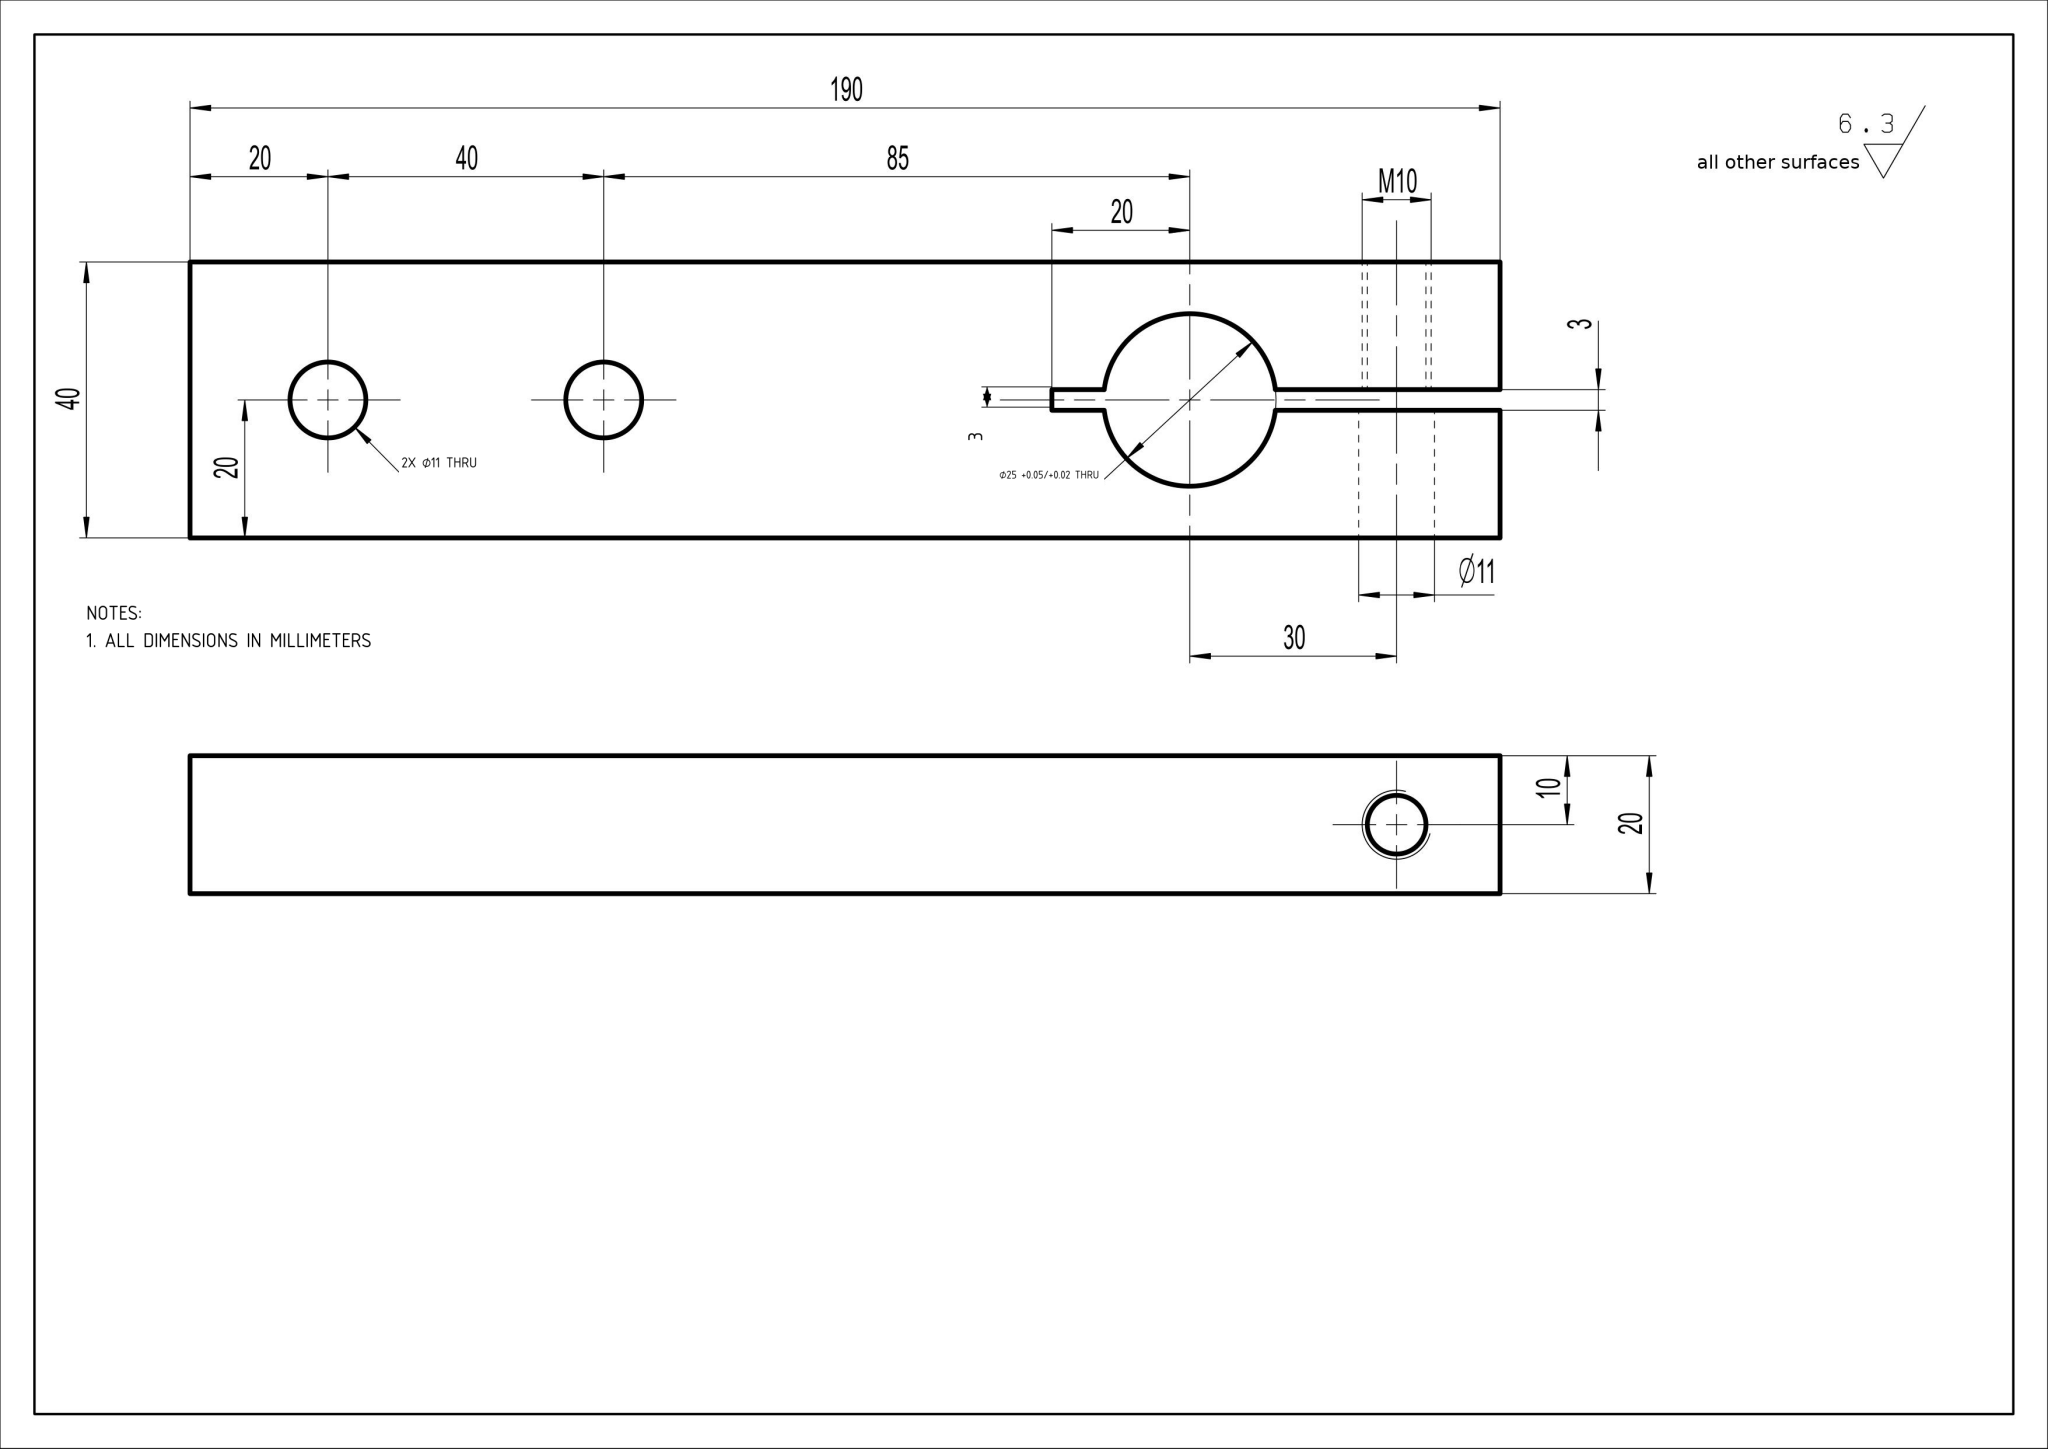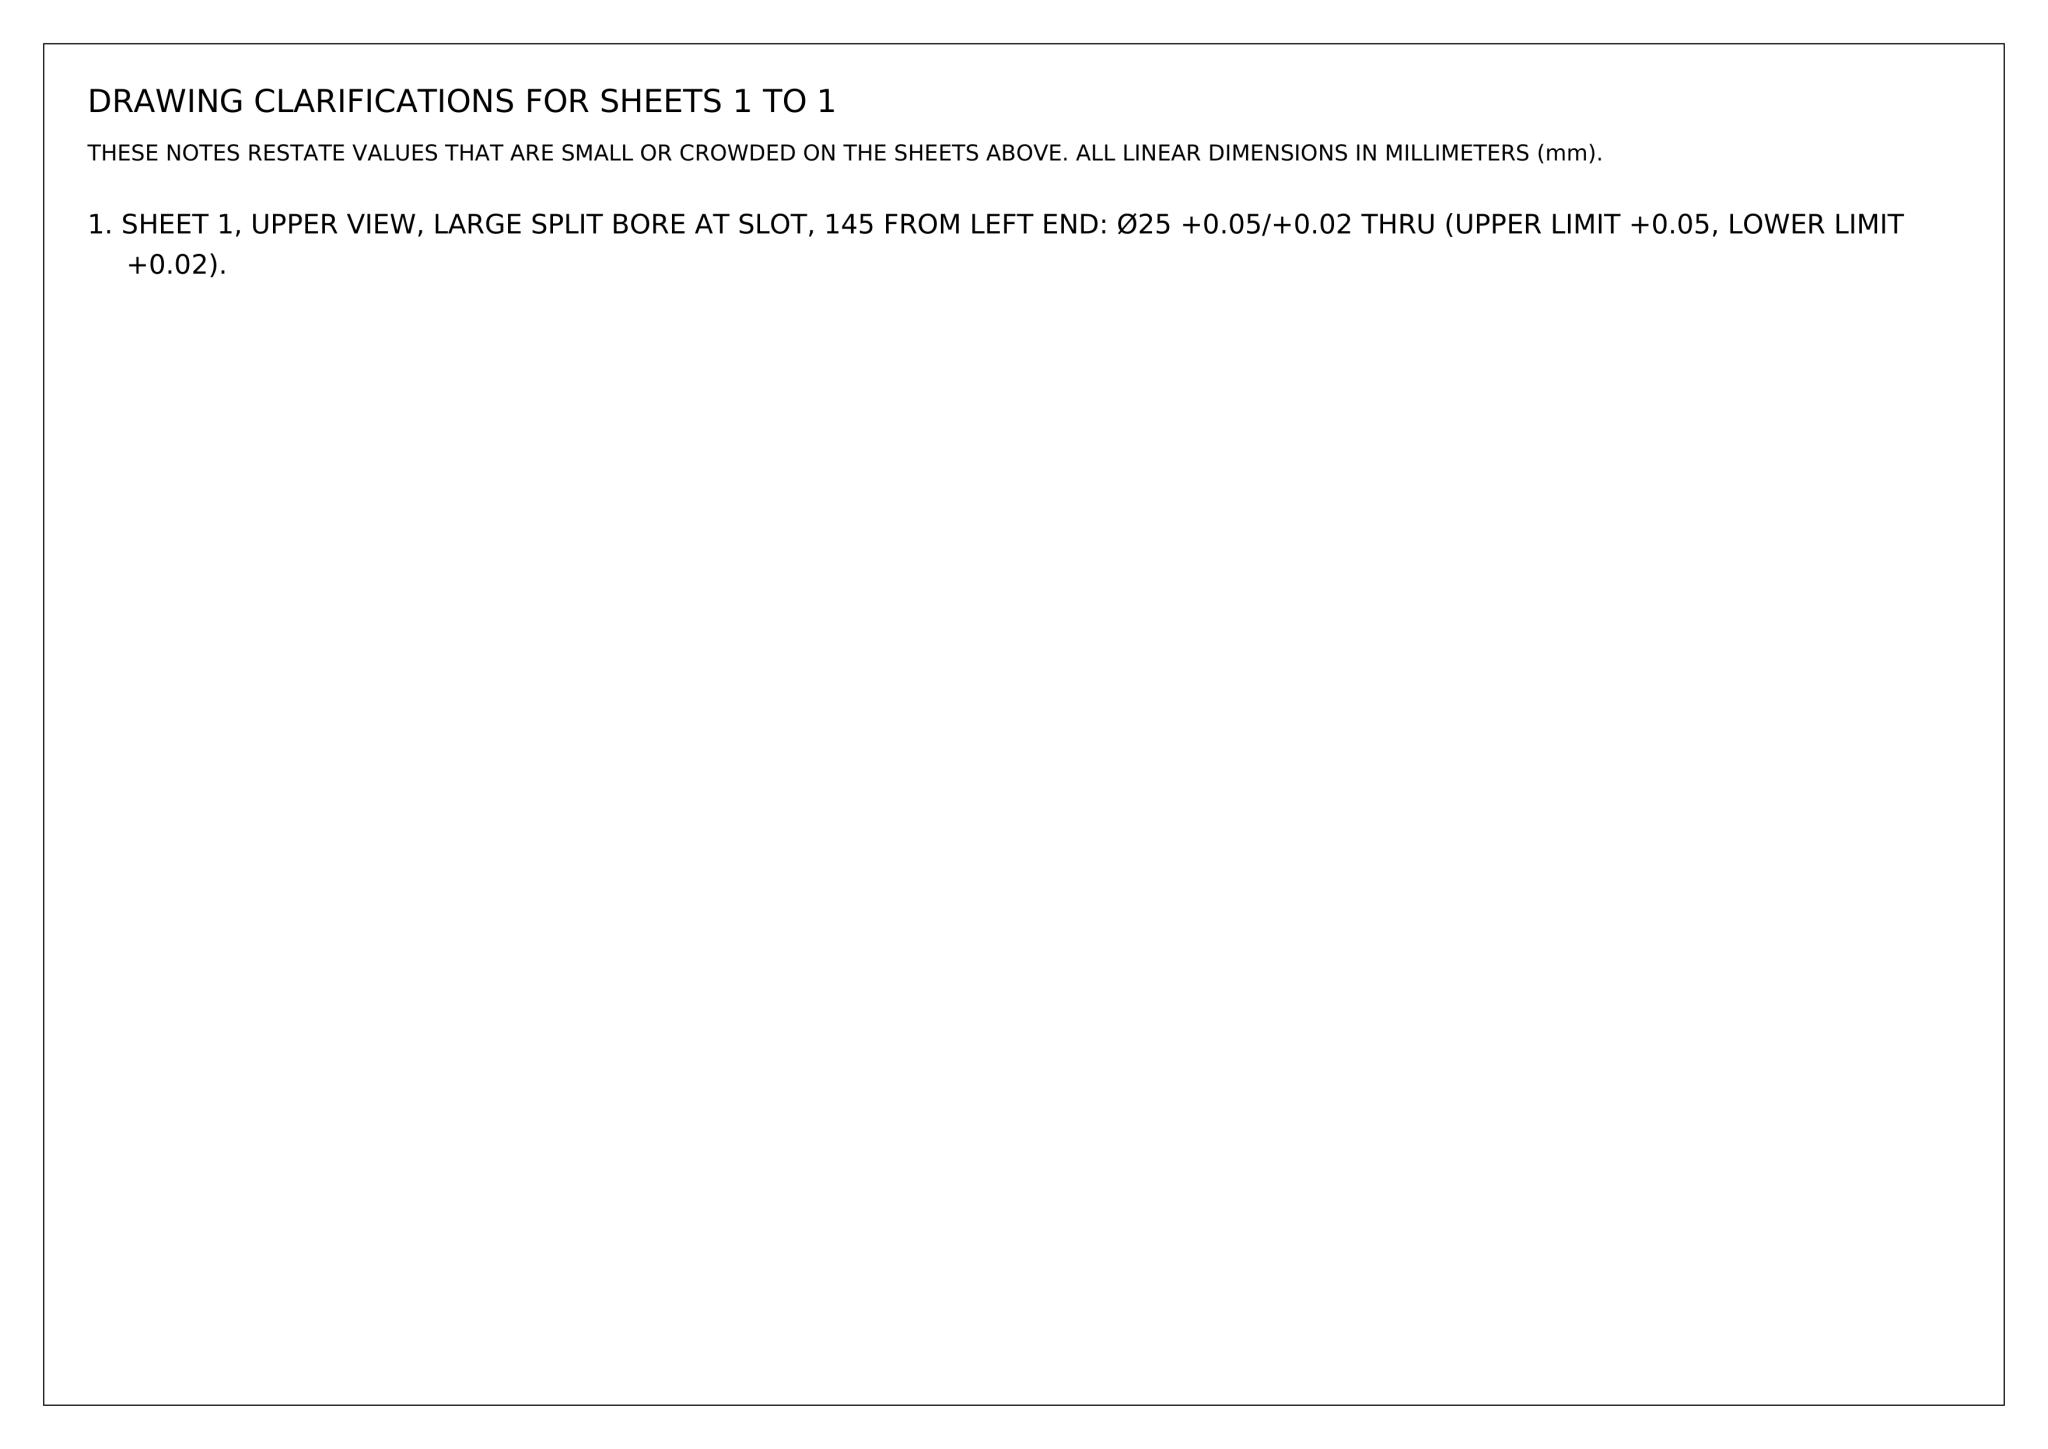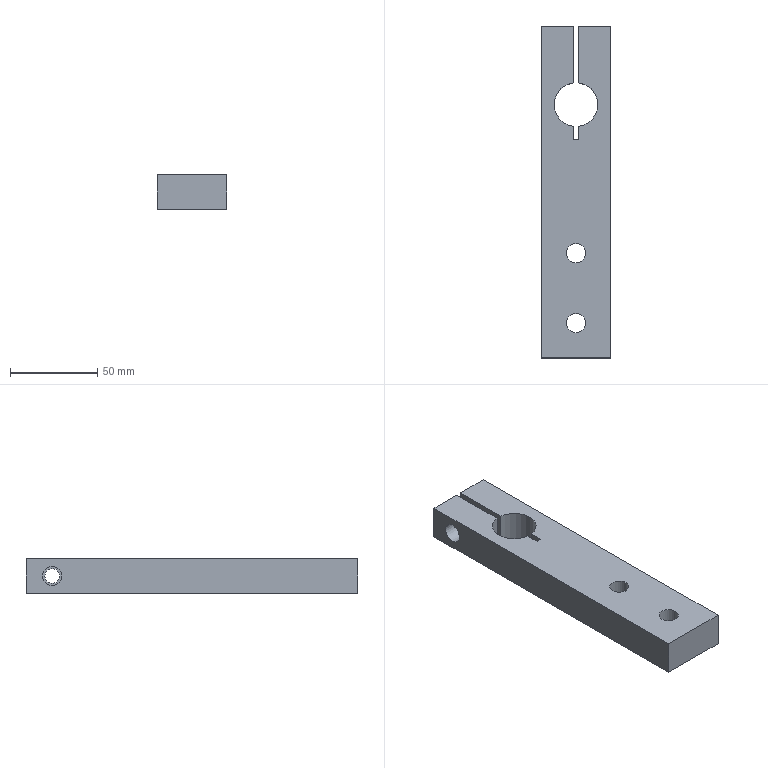Part | NX | mm | 1 solid | 18 faces | box 40 x 190 x 20 mm | volume 133170 mm3 | plane 12 | cylinder 6 | commonest cylinder face diameters 11 x3 25 x2 8.5 x1
STEP:
#1=CARTESIAN_POINT('',(0.,0.,0.));
#2=DIRECTION('',(0.,0.,1.));
#3=DIRECTION('',(1.,0.,0.));
#4=AXIS2_PLACEMENT_3D('',#1,#2,#3);
#5=(LENGTH_UNIT()NAMED_UNIT(*)SI_UNIT(.MILLI.,.METRE.));
#6=UNCERTAINTY_MEASURE_WITH_UNIT(LENGTH_MEASURE(0.00002),#5,'','');
#7=(NAMED_UNIT(*)PLANE_ANGLE_UNIT()SI_UNIT($,.RADIAN.));
#8=PLANE_ANGLE_MEASURE_WITH_UNIT(PLANE_ANGLE_MEASURE(0.01745),#7);
#9=DIMENSIONAL_EXPONENTS(0.,0.,0.,0.,0.,0.,0.);
#10=(CONVERSION_BASED_UNIT('',#8)NAMED_UNIT(#9)PLANE_ANGLE_UNIT());
#11=(NAMED_UNIT(*)SI_UNIT($,.STERADIAN.)SOLID_ANGLE_UNIT());
#12=(GEOMETRIC_REPRESENTATION_CONTEXT(3)GLOBAL_UNCERTAINTY_ASSIGNED_CONTEXT((#6))GLOBAL_UNIT_ASSIGNED_CONTEXT((#5,#10,#11))REPRESENTATION_CONTEXT('',''));
#13=SHAPE_REPRESENTATION('',(#4),#12);
#14=CARTESIAN_POINT('',(18.5,190.,0.));
#15=VERTEX_POINT('',#14);
#16=CARTESIAN_POINT('',(18.5,190.,20.));
#17=VERTEX_POINT('',#16);
#18=CARTESIAN_POINT('',(18.5,190.,-11.));
#19=DIRECTION('',(0.,0.,1.));
#20=VECTOR('',#19,1.);
#21=LINE('',#18,#20);
#22=EDGE_CURVE('',#15,#17,#21,.T.);
#23=ORIENTED_EDGE('',*,*,#22,.F.);
#24=CARTESIAN_POINT('',(-0.,190.,0.));
#25=VERTEX_POINT('',#24);
#26=CARTESIAN_POINT('',(40.,190.,0.));
#27=DIRECTION('',(-1.,0.,0.));
#28=VECTOR('',#27,1.);
#29=LINE('',#26,#28);
#30=EDGE_CURVE('',#15,#25,#29,.T.);
#31=ORIENTED_EDGE('',*,*,#30,.T.);
#32=CARTESIAN_POINT('',(-0.,190.,20.));
#33=VERTEX_POINT('',#32);
#34=CARTESIAN_POINT('',(-0.,190.,20.));
#35=DIRECTION('',(0.,0.,-1.));
#36=VECTOR('',#35,1.);
#37=LINE('',#34,#36);
#38=EDGE_CURVE('',#33,#25,#37,.T.);
#39=ORIENTED_EDGE('',*,*,#38,.F.);
#40=CARTESIAN_POINT('',(40.,190.,20.));
#41=DIRECTION('',(-1.,0.,0.));
#42=VECTOR('',#41,1.);
#43=LINE('',#40,#42);
#44=EDGE_CURVE('',#17,#33,#43,.T.);
#45=ORIENTED_EDGE('',*,*,#44,.F.);
#46=EDGE_LOOP('',(#23,#31,#39,#45));
#47=FACE_OUTER_BOUND('',#46,.T.);
#48=CARTESIAN_POINT('',(40.,190.,20.));
#49=DIRECTION('',(0.,-1.,0.));
#50=DIRECTION('',(0.,0.,-1.));
#51=AXIS2_PLACEMENT_3D('',#48,#49,#50);
#52=PLANE('',#51);
#53=ADVANCED_FACE('',(#47),#52,.F.);
#54=CARTESIAN_POINT('',(18.5,157.41,20.));
#55=VERTEX_POINT('',#54);
#56=CARTESIAN_POINT('',(18.5,157.41,0.));
#57=VERTEX_POINT('',#56);
#58=CARTESIAN_POINT('',(18.5,157.41,20.));
#59=DIRECTION('',(0.,0.,-1.));
#60=VECTOR('',#59,1.);
#61=LINE('',#58,#60);
#62=EDGE_CURVE('',#55,#57,#61,.T.);
#63=ORIENTED_EDGE('',*,*,#62,.F.);
#64=CARTESIAN_POINT('',(18.5,132.59,20.));
#65=VERTEX_POINT('',#64);
#66=CARTESIAN_POINT('',(20.,145.,20.));
#67=DIRECTION('',(0.,0.,1.));
#68=DIRECTION('',(1.,0.,0.));
#69=AXIS2_PLACEMENT_3D('',#66,#67,#68);
#70=CIRCLE('',#69,12.5);
#71=EDGE_CURVE('',#55,#65,#70,.T.);
#72=ORIENTED_EDGE('',*,*,#71,.T.);
#73=CARTESIAN_POINT('',(18.5,132.59,0.));
#74=VERTEX_POINT('',#73);
#75=CARTESIAN_POINT('',(18.5,132.59,20.));
#76=DIRECTION('',(0.,0.,1.));
#77=VECTOR('',#76,1.);
#78=LINE('',#75,#77);
#79=EDGE_CURVE('',#74,#65,#78,.T.);
#80=ORIENTED_EDGE('',*,*,#79,.F.);
#81=CARTESIAN_POINT('',(20.,145.,0.));
#82=DIRECTION('',(0.,0.,1.));
#83=DIRECTION('',(1.,0.,0.));
#84=AXIS2_PLACEMENT_3D('',#81,#82,#83);
#85=CIRCLE('',#84,12.5);
#86=EDGE_CURVE('',#57,#74,#85,.T.);
#87=ORIENTED_EDGE('',*,*,#86,.F.);
#88=EDGE_LOOP('',(#63,#72,#80,#87));
#89=FACE_OUTER_BOUND('',#88,.T.);
#90=CARTESIAN_POINT('',(20.,145.,20.));
#91=DIRECTION('',(0.,0.,-1.));
#92=DIRECTION('',(-1.,0.,0.));
#93=AXIS2_PLACEMENT_3D('',#90,#91,#92);
#94=CYLINDRICAL_SURFACE('',#93,12.5);
#95=ADVANCED_FACE('',(#89),#94,.F.);
#96=CARTESIAN_POINT('',(0.,180.5,10.));
#97=VERTEX_POINT('',#96);
#98=CARTESIAN_POINT('',(0.,175.,10.));
#99=DIRECTION('',(-1.,-0.,0.));
#100=DIRECTION('',(-0.,1.,0.));
#101=AXIS2_PLACEMENT_3D('',#98,#99,#100);
#102=CIRCLE('',#101,5.5);
#103=EDGE_CURVE('',#97,#97,#102,.T.);
#104=ORIENTED_EDGE('',*,*,#103,.F.);
#105=EDGE_LOOP('',(#104));
#106=FACE_BOUND('',#105,.T.);
#107=CARTESIAN_POINT('',(0.,0.,0.));
#108=VERTEX_POINT('',#107);
#109=CARTESIAN_POINT('',(-0.,190.,0.));
#110=DIRECTION('',(0.,-1.,0.));
#111=VECTOR('',#110,1.);
#112=LINE('',#109,#111);
#113=EDGE_CURVE('',#25,#108,#112,.T.);
#114=ORIENTED_EDGE('',*,*,#113,.T.);
#115=CARTESIAN_POINT('',(0.,0.,20.));
#116=VERTEX_POINT('',#115);
#117=CARTESIAN_POINT('',(0.,0.,20.));
#118=DIRECTION('',(0.,0.,-1.));
#119=VECTOR('',#118,1.);
#120=LINE('',#117,#119);
#121=EDGE_CURVE('',#116,#108,#120,.T.);
#122=ORIENTED_EDGE('',*,*,#121,.F.);
#123=CARTESIAN_POINT('',(-0.,190.,20.));
#124=DIRECTION('',(0.,-1.,0.));
#125=VECTOR('',#124,1.);
#126=LINE('',#123,#125);
#127=EDGE_CURVE('',#33,#116,#126,.T.);
#128=ORIENTED_EDGE('',*,*,#127,.F.);
#129=ORIENTED_EDGE('',*,*,#38,.T.);
#130=EDGE_LOOP('',(#114,#122,#128,#129));
#131=FACE_BOUND('',#130,.T.);
#132=CARTESIAN_POINT('',(-0.,190.,20.));
#133=DIRECTION('',(1.,0.,0.));
#134=DIRECTION('',(-0.,1.,0.));
#135=AXIS2_PLACEMENT_3D('',#132,#133,#134);
#136=PLANE('',#135);
#137=ADVANCED_FACE('',(#106,#131),#136,.F.);
#138=CARTESIAN_POINT('',(40.,0.,0.));
#139=VERTEX_POINT('',#138);
#140=CARTESIAN_POINT('',(0.,0.,0.));
#141=DIRECTION('',(1.,0.,0.));
#142=VECTOR('',#141,1.);
#143=LINE('',#140,#142);
#144=EDGE_CURVE('',#108,#139,#143,.T.);
#145=ORIENTED_EDGE('',*,*,#144,.T.);
#146=CARTESIAN_POINT('',(40.,0.,20.));
#147=VERTEX_POINT('',#146);
#148=CARTESIAN_POINT('',(40.,0.,20.));
#149=DIRECTION('',(0.,0.,-1.));
#150=VECTOR('',#149,1.);
#151=LINE('',#148,#150);
#152=EDGE_CURVE('',#147,#139,#151,.T.);
#153=ORIENTED_EDGE('',*,*,#152,.F.);
#154=CARTESIAN_POINT('',(0.,0.,20.));
#155=DIRECTION('',(1.,0.,0.));
#156=VECTOR('',#155,1.);
#157=LINE('',#154,#156);
#158=EDGE_CURVE('',#116,#147,#157,.T.);
#159=ORIENTED_EDGE('',*,*,#158,.F.);
#160=ORIENTED_EDGE('',*,*,#121,.T.);
#161=EDGE_LOOP('',(#145,#153,#159,#160));
#162=FACE_OUTER_BOUND('',#161,.T.);
#163=CARTESIAN_POINT('',(0.,0.,20.));
#164=DIRECTION('',(0.,1.,0.));
#165=DIRECTION('',(0.,0.,1.));
#166=AXIS2_PLACEMENT_3D('',#163,#164,#165);
#167=PLANE('',#166);
#168=ADVANCED_FACE('',(#162),#167,.F.);
#169=CARTESIAN_POINT('',(40.,170.75,10.));
#170=VERTEX_POINT('',#169);
#171=CARTESIAN_POINT('',(40.,175.,10.));
#172=DIRECTION('',(-1.,-0.,0.));
#173=DIRECTION('',(0.,-1.,0.));
#174=AXIS2_PLACEMENT_3D('',#171,#172,#173);
#175=CIRCLE('',#174,4.25);
#176=EDGE_CURVE('',#170,#170,#175,.T.);
#177=ORIENTED_EDGE('',*,*,#176,.T.);
#178=EDGE_LOOP('',(#177));
#179=FACE_BOUND('',#178,.T.);
#180=CARTESIAN_POINT('',(40.,190.,0.));
#181=VERTEX_POINT('',#180);
#182=CARTESIAN_POINT('',(40.,0.,0.));
#183=DIRECTION('',(-0.,1.,0.));
#184=VECTOR('',#183,1.);
#185=LINE('',#182,#184);
#186=EDGE_CURVE('',#139,#181,#185,.T.);
#187=ORIENTED_EDGE('',*,*,#186,.T.);
#188=CARTESIAN_POINT('',(40.,190.,20.));
#189=VERTEX_POINT('',#188);
#190=CARTESIAN_POINT('',(40.,190.,20.));
#191=DIRECTION('',(0.,0.,-1.));
#192=VECTOR('',#191,1.);
#193=LINE('',#190,#192);
#194=EDGE_CURVE('',#189,#181,#193,.T.);
#195=ORIENTED_EDGE('',*,*,#194,.F.);
#196=CARTESIAN_POINT('',(40.,0.,20.));
#197=DIRECTION('',(-0.,1.,0.));
#198=VECTOR('',#197,1.);
#199=LINE('',#196,#198);
#200=EDGE_CURVE('',#147,#189,#199,.T.);
#201=ORIENTED_EDGE('',*,*,#200,.F.);
#202=ORIENTED_EDGE('',*,*,#152,.T.);
#203=EDGE_LOOP('',(#187,#195,#201,#202));
#204=FACE_BOUND('',#203,.T.);
#205=CARTESIAN_POINT('',(40.,0.,20.));
#206=DIRECTION('',(-1.,-0.,0.));
#207=DIRECTION('',(0.,-1.,0.));
#208=AXIS2_PLACEMENT_3D('',#205,#206,#207);
#209=PLANE('',#208);
#210=ADVANCED_FACE('',(#179,#204),#209,.F.);
#211=CARTESIAN_POINT('',(25.5,20.,20.));
#212=VERTEX_POINT('',#211);
#213=CARTESIAN_POINT('',(20.,20.,20.));
#214=DIRECTION('',(0.,0.,1.));
#215=DIRECTION('',(1.,0.,0.));
#216=AXIS2_PLACEMENT_3D('',#213,#214,#215);
#217=CIRCLE('',#216,5.5);
#218=EDGE_CURVE('',#212,#212,#217,.T.);
#219=ORIENTED_EDGE('',*,*,#218,.T.);
#220=EDGE_LOOP('',(#219));
#221=FACE_BOUND('',#220,.T.);
#222=CARTESIAN_POINT('',(25.5,20.,0.));
#223=VERTEX_POINT('',#222);
#224=CARTESIAN_POINT('',(20.,20.,0.));
#225=DIRECTION('',(0.,0.,1.));
#226=DIRECTION('',(1.,0.,0.));
#227=AXIS2_PLACEMENT_3D('',#224,#225,#226);
#228=CIRCLE('',#227,5.5);
#229=EDGE_CURVE('',#223,#223,#228,.T.);
#230=ORIENTED_EDGE('',*,*,#229,.F.);
#231=EDGE_LOOP('',(#230));
#232=FACE_BOUND('',#231,.T.);
#233=CARTESIAN_POINT('',(20.,20.,20.));
#234=DIRECTION('',(0.,0.,-1.));
#235=DIRECTION('',(-1.,0.,0.));
#236=AXIS2_PLACEMENT_3D('',#233,#234,#235);
#237=CYLINDRICAL_SURFACE('',#236,5.5);
#238=ADVANCED_FACE('',(#221,#232),#237,.F.);
#239=CARTESIAN_POINT('',(21.5,132.59,20.));
#240=VERTEX_POINT('',#239);
#241=CARTESIAN_POINT('',(21.5,132.59,0.));
#242=VERTEX_POINT('',#241);
#243=CARTESIAN_POINT('',(21.5,132.59,20.));
#244=DIRECTION('',(0.,0.,-1.));
#245=VECTOR('',#244,1.);
#246=LINE('',#243,#245);
#247=EDGE_CURVE('',#240,#242,#246,.T.);
#248=ORIENTED_EDGE('',*,*,#247,.F.);
#249=CARTESIAN_POINT('',(21.5,157.41,20.));
#250=VERTEX_POINT('',#249);
#251=CARTESIAN_POINT('',(20.,145.,20.));
#252=DIRECTION('',(0.,0.,1.));
#253=DIRECTION('',(1.,0.,0.));
#254=AXIS2_PLACEMENT_3D('',#251,#252,#253);
#255=CIRCLE('',#254,12.5);
#256=EDGE_CURVE('',#240,#250,#255,.T.);
#257=ORIENTED_EDGE('',*,*,#256,.T.);
#258=CARTESIAN_POINT('',(21.5,157.41,0.));
#259=VERTEX_POINT('',#258);
#260=CARTESIAN_POINT('',(21.5,157.41,20.));
#261=DIRECTION('',(0.,0.,1.));
#262=VECTOR('',#261,1.);
#263=LINE('',#260,#262);
#264=EDGE_CURVE('',#259,#250,#263,.T.);
#265=ORIENTED_EDGE('',*,*,#264,.F.);
#266=CARTESIAN_POINT('',(20.,145.,0.));
#267=DIRECTION('',(0.,0.,1.));
#268=DIRECTION('',(1.,0.,0.));
#269=AXIS2_PLACEMENT_3D('',#266,#267,#268);
#270=CIRCLE('',#269,12.5);
#271=EDGE_CURVE('',#242,#259,#270,.T.);
#272=ORIENTED_EDGE('',*,*,#271,.F.);
#273=EDGE_LOOP('',(#248,#257,#265,#272));
#274=FACE_OUTER_BOUND('',#273,.T.);
#275=CARTESIAN_POINT('',(20.,145.,20.));
#276=DIRECTION('',(0.,0.,-1.));
#277=DIRECTION('',(-1.,0.,0.));
#278=AXIS2_PLACEMENT_3D('',#275,#276,#277);
#279=CYLINDRICAL_SURFACE('',#278,12.5);
#280=ADVANCED_FACE('',(#274),#279,.F.);
#281=CARTESIAN_POINT('',(21.5,190.,0.));
#282=VERTEX_POINT('',#281);
#283=CARTESIAN_POINT('',(40.,190.,0.));
#284=DIRECTION('',(-1.,0.,0.));
#285=VECTOR('',#284,1.);
#286=LINE('',#283,#285);
#287=EDGE_CURVE('',#181,#282,#286,.T.);
#288=ORIENTED_EDGE('',*,*,#287,.T.);
#289=CARTESIAN_POINT('',(21.5,190.,20.));
#290=VERTEX_POINT('',#289);
#291=CARTESIAN_POINT('',(21.5,190.,-11.));
#292=DIRECTION('',(0.,0.,1.));
#293=VECTOR('',#292,1.);
#294=LINE('',#291,#293);
#295=EDGE_CURVE('',#282,#290,#294,.T.);
#296=ORIENTED_EDGE('',*,*,#295,.T.);
#297=CARTESIAN_POINT('',(40.,190.,20.));
#298=DIRECTION('',(-1.,0.,0.));
#299=VECTOR('',#298,1.);
#300=LINE('',#297,#299);
#301=EDGE_CURVE('',#189,#290,#300,.T.);
#302=ORIENTED_EDGE('',*,*,#301,.F.);
#303=ORIENTED_EDGE('',*,*,#194,.T.);
#304=EDGE_LOOP('',(#288,#296,#302,#303));
#305=FACE_OUTER_BOUND('',#304,.T.);
#306=CARTESIAN_POINT('',(40.,190.,20.));
#307=DIRECTION('',(0.,-1.,0.));
#308=DIRECTION('',(0.,0.,-1.));
#309=AXIS2_PLACEMENT_3D('',#306,#307,#308);
#310=PLANE('',#309);
#311=ADVANCED_FACE('',(#305),#310,.F.);
#312=CARTESIAN_POINT('',(25.5,60.,20.));
#313=VERTEX_POINT('',#312);
#314=CARTESIAN_POINT('',(20.,60.,20.));
#315=DIRECTION('',(0.,0.,1.));
#316=DIRECTION('',(1.,0.,0.));
#317=AXIS2_PLACEMENT_3D('',#314,#315,#316);
#318=CIRCLE('',#317,5.5);
#319=EDGE_CURVE('',#313,#313,#318,.T.);
#320=ORIENTED_EDGE('',*,*,#319,.T.);
#321=EDGE_LOOP('',(#320));
#322=FACE_BOUND('',#321,.T.);
#323=CARTESIAN_POINT('',(25.5,60.,0.));
#324=VERTEX_POINT('',#323);
#325=CARTESIAN_POINT('',(20.,60.,0.));
#326=DIRECTION('',(0.,0.,1.));
#327=DIRECTION('',(1.,0.,0.));
#328=AXIS2_PLACEMENT_3D('',#325,#326,#327);
#329=CIRCLE('',#328,5.5);
#330=EDGE_CURVE('',#324,#324,#329,.T.);
#331=ORIENTED_EDGE('',*,*,#330,.F.);
#332=EDGE_LOOP('',(#331));
#333=FACE_BOUND('',#332,.T.);
#334=CARTESIAN_POINT('',(20.,60.,20.));
#335=DIRECTION('',(0.,0.,-1.));
#336=DIRECTION('',(-1.,0.,0.));
#337=AXIS2_PLACEMENT_3D('',#334,#335,#336);
#338=CYLINDRICAL_SURFACE('',#337,5.5);
#339=ADVANCED_FACE('',(#322,#333),#338,.F.);
#340=CARTESIAN_POINT('',(18.5,190.,20.));
#341=DIRECTION('',(-0.,-1.,0.));
#342=VECTOR('',#341,1.);
#343=LINE('',#340,#342);
#344=EDGE_CURVE('',#17,#55,#343,.T.);
#345=ORIENTED_EDGE('',*,*,#344,.F.);
#346=ORIENTED_EDGE('',*,*,#44,.T.);
#347=ORIENTED_EDGE('',*,*,#127,.T.);
#348=ORIENTED_EDGE('',*,*,#158,.T.);
#349=ORIENTED_EDGE('',*,*,#200,.T.);
#350=ORIENTED_EDGE('',*,*,#301,.T.);
#351=CARTESIAN_POINT('',(21.5,125.,20.));
#352=DIRECTION('',(-0.,1.,0.));
#353=VECTOR('',#352,1.);
#354=LINE('',#351,#353);
#355=EDGE_CURVE('',#250,#290,#354,.T.);
#356=ORIENTED_EDGE('',*,*,#355,.F.);
#357=ORIENTED_EDGE('',*,*,#256,.F.);
#358=CARTESIAN_POINT('',(21.5,125.,20.));
#359=VERTEX_POINT('',#358);
#360=CARTESIAN_POINT('',(21.5,125.,20.));
#361=DIRECTION('',(-0.,1.,0.));
#362=VECTOR('',#361,1.);
#363=LINE('',#360,#362);
#364=EDGE_CURVE('',#359,#240,#363,.T.);
#365=ORIENTED_EDGE('',*,*,#364,.F.);
#366=CARTESIAN_POINT('',(18.5,125.,20.));
#367=VERTEX_POINT('',#366);
#368=CARTESIAN_POINT('',(18.5,125.,20.));
#369=DIRECTION('',(1.,0.,0.));
#370=VECTOR('',#369,1.);
#371=LINE('',#368,#370);
#372=EDGE_CURVE('',#367,#359,#371,.T.);
#373=ORIENTED_EDGE('',*,*,#372,.F.);
#374=CARTESIAN_POINT('',(18.5,190.,20.));
#375=DIRECTION('',(-0.,-1.,0.));
#376=VECTOR('',#375,1.);
#377=LINE('',#374,#376);
#378=EDGE_CURVE('',#65,#367,#377,.T.);
#379=ORIENTED_EDGE('',*,*,#378,.F.);
#380=ORIENTED_EDGE('',*,*,#71,.F.);
#381=EDGE_LOOP('',(#345,#346,#347,#348,#349,#350,#356,#357,#365,#373,#379,#380));
#382=FACE_BOUND('',#381,.T.);
#383=ORIENTED_EDGE('',*,*,#218,.F.);
#384=EDGE_LOOP('',(#383));
#385=FACE_BOUND('',#384,.T.);
#386=ORIENTED_EDGE('',*,*,#319,.F.);
#387=EDGE_LOOP('',(#386));
#388=FACE_BOUND('',#387,.T.);
#389=CARTESIAN_POINT('',(20.,145.,20.));
#390=DIRECTION('',(0.,0.,1.));
#391=DIRECTION('',(1.,0.,0.));
#392=AXIS2_PLACEMENT_3D('',#389,#390,#391);
#393=PLANE('',#392);
#394=ADVANCED_FACE('',(#382,#385,#388),#393,.T.);
#395=ORIENTED_EDGE('',*,*,#30,.F.);
#396=CARTESIAN_POINT('',(18.5,145.,0.));
#397=DIRECTION('',(-0.,-1.,0.));
#398=VECTOR('',#397,1.);
#399=LINE('',#396,#398);
#400=EDGE_CURVE('',#15,#57,#399,.T.);
#401=ORIENTED_EDGE('',*,*,#400,.T.);
#402=ORIENTED_EDGE('',*,*,#86,.T.);
#403=CARTESIAN_POINT('',(18.5,125.,0.));
#404=VERTEX_POINT('',#403);
#405=CARTESIAN_POINT('',(18.5,145.,0.));
#406=DIRECTION('',(-0.,-1.,0.));
#407=VECTOR('',#406,1.);
#408=LINE('',#405,#407);
#409=EDGE_CURVE('',#74,#404,#408,.T.);
#410=ORIENTED_EDGE('',*,*,#409,.T.);
#411=CARTESIAN_POINT('',(21.5,125.,0.));
#412=VERTEX_POINT('',#411);
#413=CARTESIAN_POINT('',(20.,125.,0.));
#414=DIRECTION('',(1.,0.,0.));
#415=VECTOR('',#414,1.);
#416=LINE('',#413,#415);
#417=EDGE_CURVE('',#404,#412,#416,.T.);
#418=ORIENTED_EDGE('',*,*,#417,.T.);
#419=CARTESIAN_POINT('',(21.5,145.,0.));
#420=DIRECTION('',(-0.,1.,0.));
#421=VECTOR('',#420,1.);
#422=LINE('',#419,#421);
#423=EDGE_CURVE('',#412,#242,#422,.T.);
#424=ORIENTED_EDGE('',*,*,#423,.T.);
#425=ORIENTED_EDGE('',*,*,#271,.T.);
#426=CARTESIAN_POINT('',(21.5,145.,0.));
#427=DIRECTION('',(-0.,1.,0.));
#428=VECTOR('',#427,1.);
#429=LINE('',#426,#428);
#430=EDGE_CURVE('',#259,#282,#429,.T.);
#431=ORIENTED_EDGE('',*,*,#430,.T.);
#432=ORIENTED_EDGE('',*,*,#287,.F.);
#433=ORIENTED_EDGE('',*,*,#186,.F.);
#434=ORIENTED_EDGE('',*,*,#144,.F.);
#435=ORIENTED_EDGE('',*,*,#113,.F.);
#436=EDGE_LOOP('',(#395,#401,#402,#410,#418,#424,#425,#431,#432,#433,#434,#435));
#437=FACE_BOUND('',#436,.T.);
#438=ORIENTED_EDGE('',*,*,#229,.T.);
#439=EDGE_LOOP('',(#438));
#440=FACE_BOUND('',#439,.T.);
#441=ORIENTED_EDGE('',*,*,#330,.T.);
#442=EDGE_LOOP('',(#441));
#443=FACE_BOUND('',#442,.T.);
#444=CARTESIAN_POINT('',(20.,145.,0.));
#445=DIRECTION('',(0.,0.,1.));
#446=DIRECTION('',(1.,0.,0.));
#447=AXIS2_PLACEMENT_3D('',#444,#445,#446);
#448=PLANE('',#447);
#449=ADVANCED_FACE('',(#437,#440,#443),#448,.F.);
#450=CARTESIAN_POINT('',(21.5,179.25,10.));
#451=VERTEX_POINT('',#450);
#452=CARTESIAN_POINT('',(21.5,175.,10.));
#453=DIRECTION('',(1.,0.,0.));
#454=DIRECTION('',(0.,1.,0.));
#455=AXIS2_PLACEMENT_3D('',#452,#453,#454);
#456=CIRCLE('',#455,4.25);
#457=EDGE_CURVE('',#451,#451,#456,.T.);
#458=ORIENTED_EDGE('',*,*,#457,.T.);
#459=EDGE_LOOP('',(#458));
#460=FACE_BOUND('',#459,.T.);
#461=ORIENTED_EDGE('',*,*,#264,.T.);
#462=ORIENTED_EDGE('',*,*,#355,.T.);
#463=ORIENTED_EDGE('',*,*,#295,.F.);
#464=ORIENTED_EDGE('',*,*,#430,.F.);
#465=EDGE_LOOP('',(#461,#462,#463,#464));
#466=FACE_BOUND('',#465,.T.);
#467=CARTESIAN_POINT('',(21.5,125.,-11.));
#468=DIRECTION('',(1.,0.,0.));
#469=DIRECTION('',(-0.,1.,0.));
#470=AXIS2_PLACEMENT_3D('',#467,#468,#469);
#471=PLANE('',#470);
#472=ADVANCED_FACE('',(#460,#466),#471,.F.);
#473=ORIENTED_EDGE('',*,*,#247,.T.);
#474=ORIENTED_EDGE('',*,*,#423,.F.);
#475=CARTESIAN_POINT('',(21.5,125.,-11.));
#476=DIRECTION('',(0.,0.,-1.));
#477=VECTOR('',#476,1.);
#478=LINE('',#475,#477);
#479=EDGE_CURVE('',#359,#412,#478,.T.);
#480=ORIENTED_EDGE('',*,*,#479,.F.);
#481=ORIENTED_EDGE('',*,*,#364,.T.);
#482=EDGE_LOOP('',(#473,#474,#480,#481));
#483=FACE_OUTER_BOUND('',#482,.T.);
#484=CARTESIAN_POINT('',(21.5,125.,-11.));
#485=DIRECTION('',(1.,0.,0.));
#486=DIRECTION('',(-0.,1.,0.));
#487=AXIS2_PLACEMENT_3D('',#484,#485,#486);
#488=PLANE('',#487);
#489=ADVANCED_FACE('',(#483),#488,.F.);
#490=CARTESIAN_POINT('',(18.5,125.,-11.));
#491=DIRECTION('',(0.,0.,-1.));
#492=VECTOR('',#491,1.);
#493=LINE('',#490,#492);
#494=EDGE_CURVE('',#367,#404,#493,.T.);
#495=ORIENTED_EDGE('',*,*,#494,.F.);
#496=ORIENTED_EDGE('',*,*,#372,.T.);
#497=ORIENTED_EDGE('',*,*,#479,.T.);
#498=ORIENTED_EDGE('',*,*,#417,.F.);
#499=EDGE_LOOP('',(#495,#496,#497,#498));
#500=FACE_OUTER_BOUND('',#499,.T.);
#501=CARTESIAN_POINT('',(18.5,125.,-11.));
#502=DIRECTION('',(0.,-1.,0.));
#503=DIRECTION('',(0.,0.,-1.));
#504=AXIS2_PLACEMENT_3D('',#501,#502,#503);
#505=PLANE('',#504);
#506=ADVANCED_FACE('',(#500),#505,.F.);
#507=ORIENTED_EDGE('',*,*,#79,.T.);
#508=ORIENTED_EDGE('',*,*,#378,.T.);
#509=ORIENTED_EDGE('',*,*,#494,.T.);
#510=ORIENTED_EDGE('',*,*,#409,.F.);
#511=EDGE_LOOP('',(#507,#508,#509,#510));
#512=FACE_OUTER_BOUND('',#511,.T.);
#513=CARTESIAN_POINT('',(18.5,190.,-11.));
#514=DIRECTION('',(-1.,0.,0.));
#515=DIRECTION('',(-0.,-1.,0.));
#516=AXIS2_PLACEMENT_3D('',#513,#514,#515);
#517=PLANE('',#516);
#518=ADVANCED_FACE('',(#512),#517,.F.);
#519=CARTESIAN_POINT('',(18.5,169.5,10.));
#520=VERTEX_POINT('',#519);
#521=CARTESIAN_POINT('',(18.5,175.,10.));
#522=DIRECTION('',(-1.,0.,0.));
#523=DIRECTION('',(0.,-1.,0.));
#524=AXIS2_PLACEMENT_3D('',#521,#522,#523);
#525=CIRCLE('',#524,5.5);
#526=EDGE_CURVE('',#520,#520,#525,.T.);
#527=ORIENTED_EDGE('',*,*,#526,.T.);
#528=EDGE_LOOP('',(#527));
#529=FACE_BOUND('',#528,.T.);
#530=ORIENTED_EDGE('',*,*,#62,.T.);
#531=ORIENTED_EDGE('',*,*,#400,.F.);
#532=ORIENTED_EDGE('',*,*,#22,.T.);
#533=ORIENTED_EDGE('',*,*,#344,.T.);
#534=EDGE_LOOP('',(#530,#531,#532,#533));
#535=FACE_BOUND('',#534,.T.);
#536=CARTESIAN_POINT('',(18.5,190.,-11.));
#537=DIRECTION('',(-1.,0.,0.));
#538=DIRECTION('',(-0.,-1.,0.));
#539=AXIS2_PLACEMENT_3D('',#536,#537,#538);
#540=PLANE('',#539);
#541=ADVANCED_FACE('',(#529,#535),#540,.F.);
#542=ORIENTED_EDGE('',*,*,#103,.T.);
#543=EDGE_LOOP('',(#542));
#544=FACE_BOUND('',#543,.T.);
#545=ORIENTED_EDGE('',*,*,#526,.F.);
#546=EDGE_LOOP('',(#545));
#547=FACE_BOUND('',#546,.T.);
#548=CARTESIAN_POINT('',(73.,175.,10.));
#549=DIRECTION('',(-1.,-0.,0.));
#550=DIRECTION('',(0.,-1.,0.));
#551=AXIS2_PLACEMENT_3D('',#548,#549,#550);
#552=CYLINDRICAL_SURFACE('',#551,5.5);
#553=ADVANCED_FACE('',(#544,#547),#552,.F.);
#554=ORIENTED_EDGE('',*,*,#457,.F.);
#555=EDGE_LOOP('',(#554));
#556=FACE_BOUND('',#555,.T.);
#557=ORIENTED_EDGE('',*,*,#176,.F.);
#558=EDGE_LOOP('',(#557));
#559=FACE_BOUND('',#558,.T.);
#560=CARTESIAN_POINT('',(73.,175.,10.));
#561=DIRECTION('',(-1.,-0.,0.));
#562=DIRECTION('',(0.,-1.,0.));
#563=AXIS2_PLACEMENT_3D('',#560,#561,#562);
#564=CYLINDRICAL_SURFACE('',#563,4.25);
#565=ADVANCED_FACE('',(#556,#559),#564,.F.);
#566=CLOSED_SHELL('',(#53,#95,#137,#168,#210,#238,#280,#311,#339,#394,#449,#472,#489,#506,#518,#541,#553,#565));
#567=MANIFOLD_SOLID_BREP('',#566);
#568=ADVANCED_BREP_SHAPE_REPRESENTATION('',(#567),#12);
#569=SHAPE_REPRESENTATION_RELATIONSHIP('','',#13,#568);
#570=PRESENTATION_LAYER_ASSIGNMENT('','',(#567));
#571=COLOUR_RGB('',0.8,0.8,0.8);
#572=FILL_AREA_STYLE_COLOUR('',#571);
#573=FILL_AREA_STYLE('',(#572));
#574=SURFACE_STYLE_FILL_AREA(#573);
#575=SURFACE_SIDE_STYLE('',(#574));
#576=SURFACE_STYLE_USAGE(.BOTH.,#575);
#577=PRESENTATION_STYLE_ASSIGNMENT((#576));
#578=STYLED_ITEM('',(#577),#567);
#579=MECHANICAL_DESIGN_GEOMETRIC_PRESENTATION_REPRESENTATION('',(#578),#12);